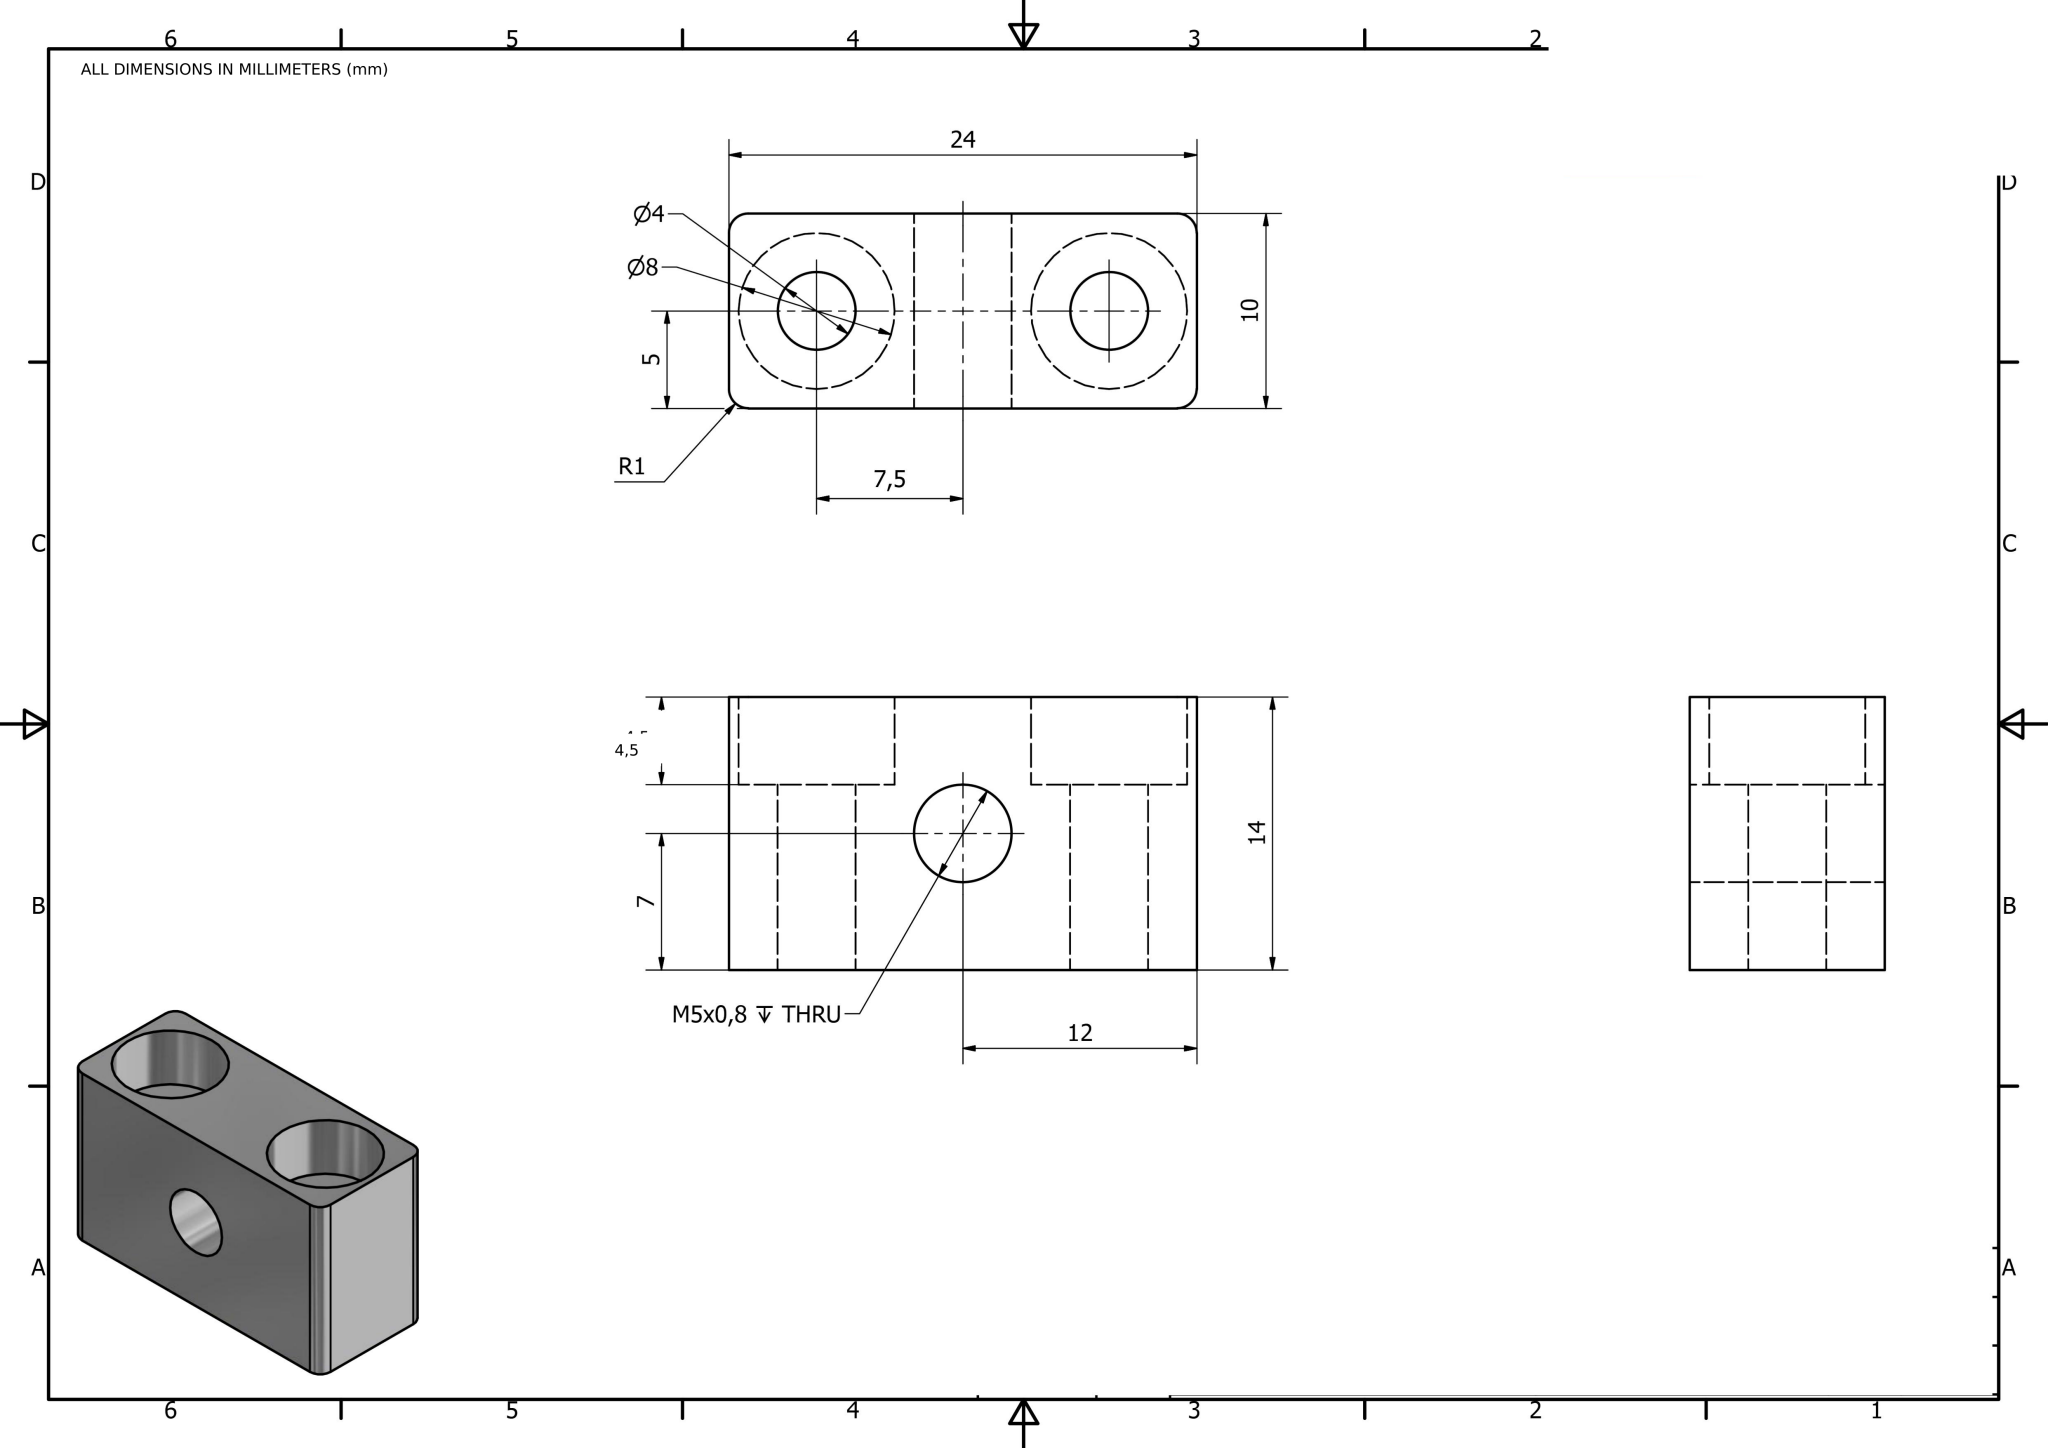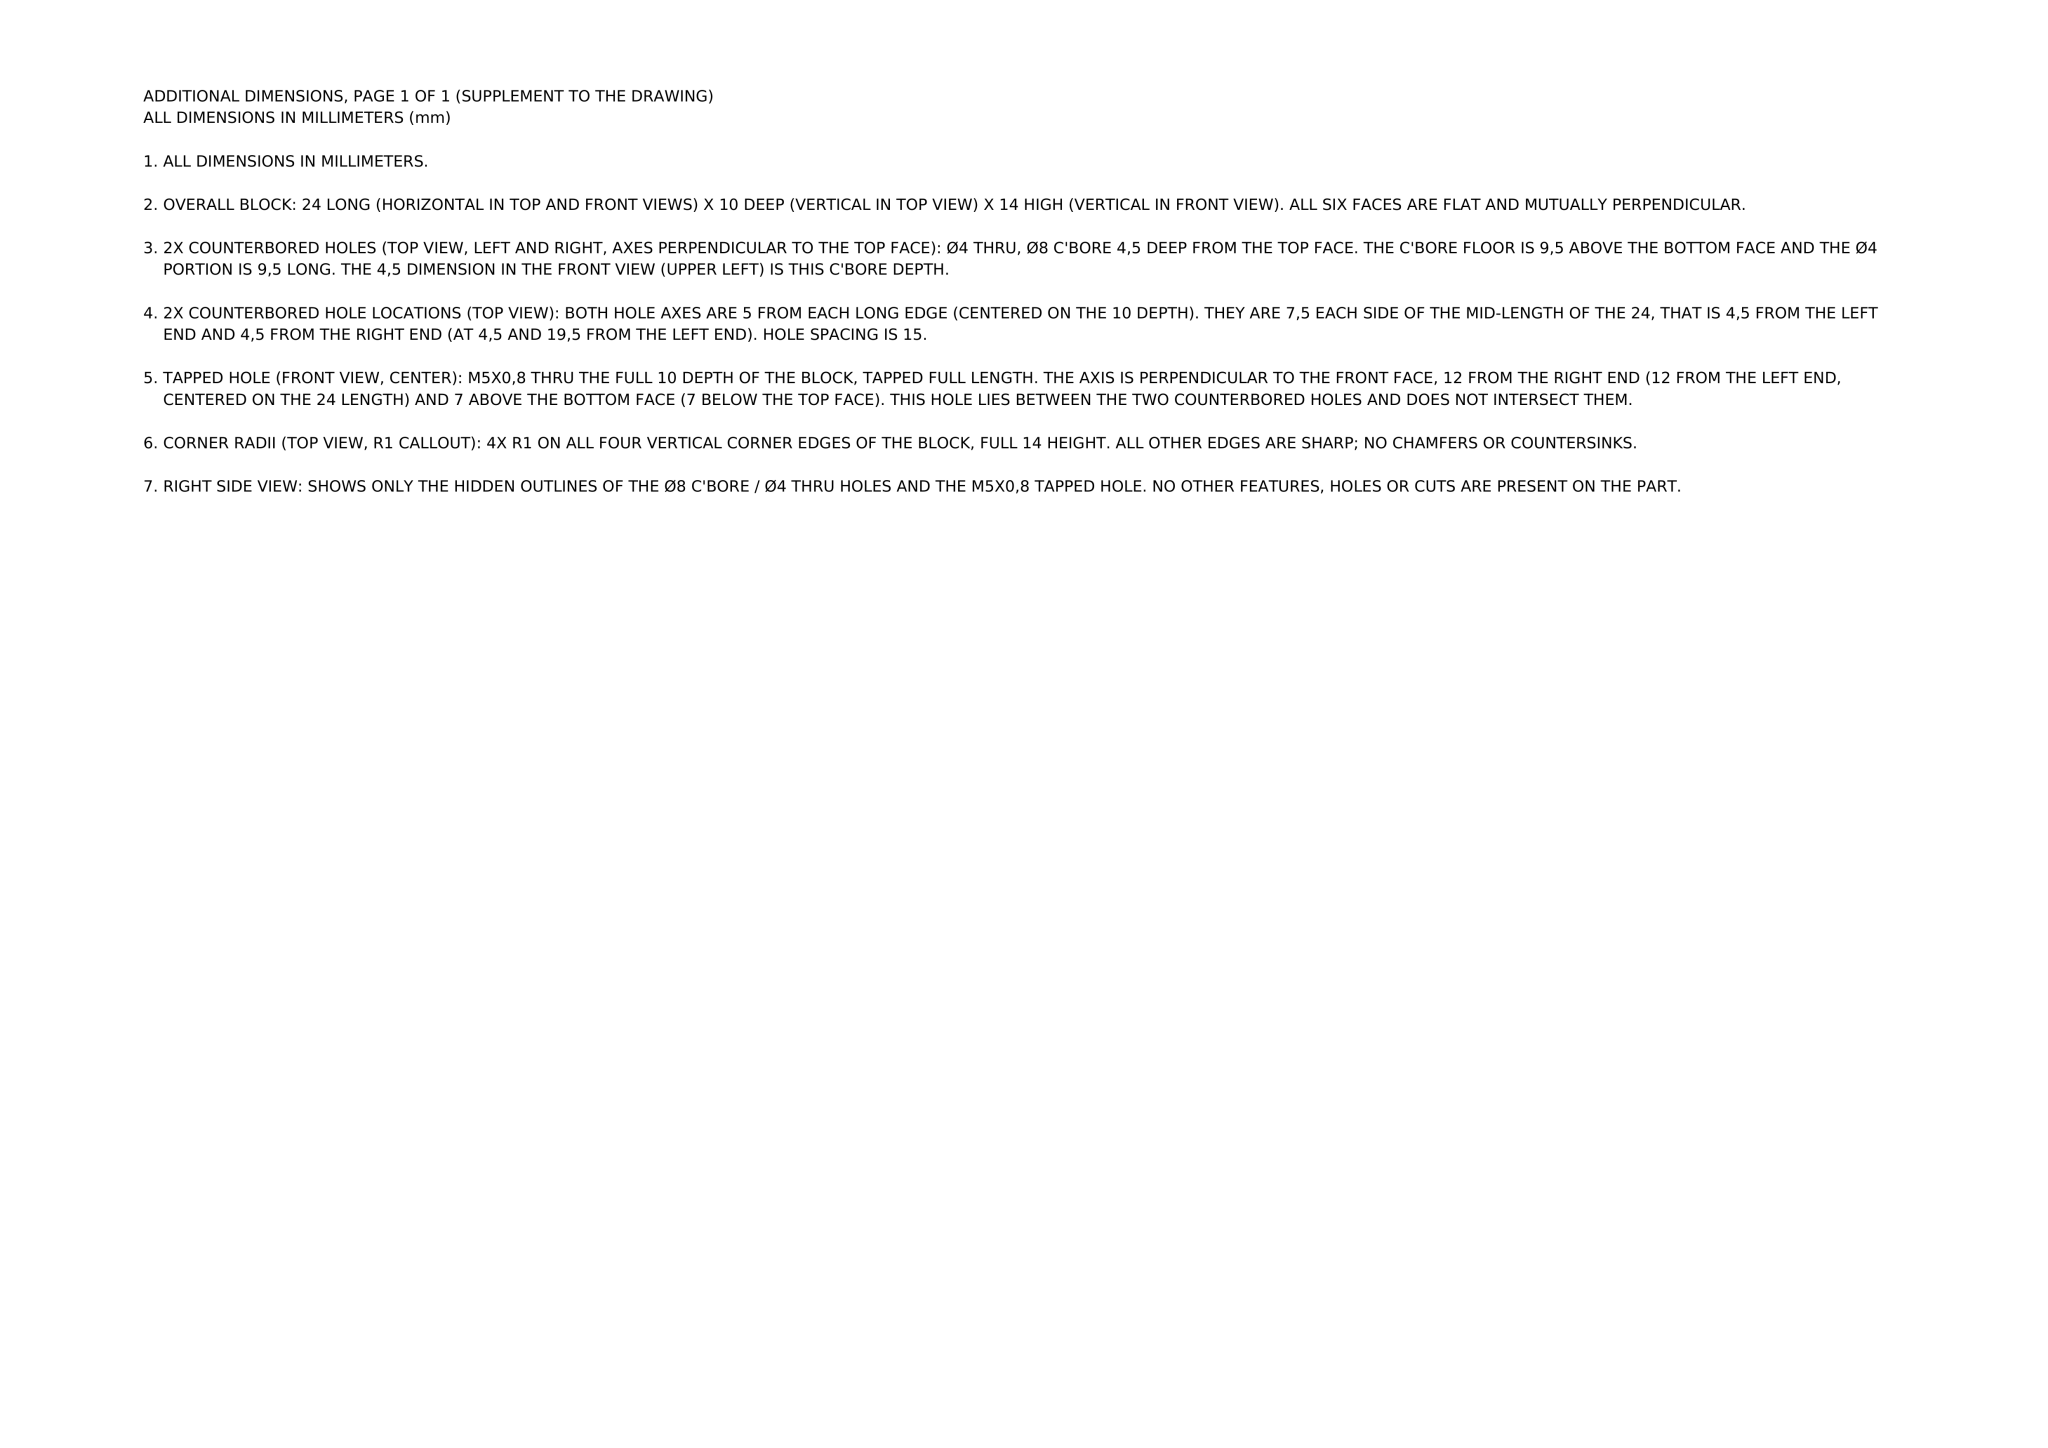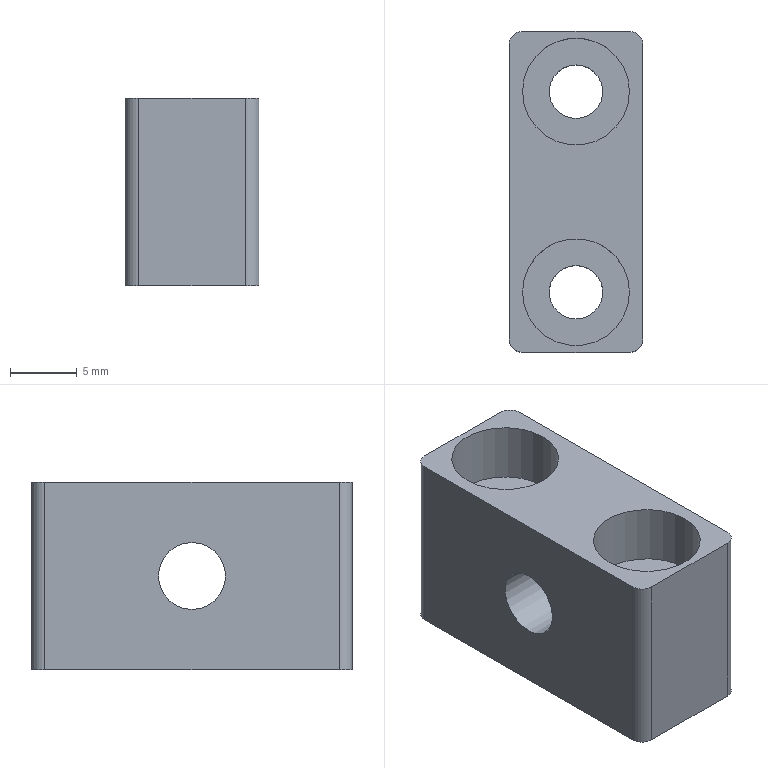Part | NX | mm | 1 solid | 17 faces | box 10 x 24 x 14 mm | volume 2460 mm3 | cylinder 9 | plane 8 | commonest cylinder face diameters 2 x4 8 x2 4 x2 5 x1
STEP:
#1=COLOUR_RGB('',0.9569,0.9569,0.9569);
#2=FILL_AREA_STYLE_COLOUR('',#1);
#3=FILL_AREA_STYLE('',(#2));
#4=SURFACE_STYLE_FILL_AREA(#3);
#5=SURFACE_SIDE_STYLE('',(#4));
#6=SURFACE_STYLE_USAGE(.BOTH.,#5);
#7=PRESENTATION_STYLE_ASSIGNMENT((#6));
#8=CARTESIAN_POINT('',(183.489,223.02,108.));
#9=VERTEX_POINT('',#8);
#10=CARTESIAN_POINT('',(182.489,222.02,108.));
#11=VERTEX_POINT('',#10);
#12=CARTESIAN_POINT('',(182.489,223.02,108.));
#13=DIRECTION('',(0.,0.,-1.));
#14=DIRECTION('',(0.7071,-0.7071,0.));
#15=AXIS2_PLACEMENT_3D('',#12,#13,#14);
#16=CIRCLE('',#15,1.);
#17=EDGE_CURVE('',#9,#11,#16,.T.);
#18=ORIENTED_EDGE('',*,*,#17,.T.);
#19=CARTESIAN_POINT('',(182.489,222.02,94.));
#20=VERTEX_POINT('',#19);
#21=CARTESIAN_POINT('',(182.489,222.02,94.));
#22=DIRECTION('',(0.,0.,-1.));
#23=VECTOR('',#22,1.);
#24=LINE('',#21,#23);
#25=EDGE_CURVE('',#11,#20,#24,.T.);
#26=ORIENTED_EDGE('',*,*,#25,.T.);
#27=CARTESIAN_POINT('',(183.489,223.02,94.));
#28=VERTEX_POINT('',#27);
#29=CARTESIAN_POINT('',(182.489,223.02,94.));
#30=DIRECTION('',(-0.,-0.,1.));
#31=DIRECTION('',(0.7071,-0.7071,0.));
#32=AXIS2_PLACEMENT_3D('',#29,#30,#31);
#33=CIRCLE('',#32,1.);
#34=EDGE_CURVE('',#20,#28,#33,.T.);
#35=ORIENTED_EDGE('',*,*,#34,.T.);
#36=CARTESIAN_POINT('',(183.489,223.02,94.));
#37=DIRECTION('',(0.,0.,1.));
#38=VECTOR('',#37,1.);
#39=LINE('',#36,#38);
#40=EDGE_CURVE('',#28,#9,#39,.T.);
#41=ORIENTED_EDGE('',*,*,#40,.T.);
#42=EDGE_LOOP('',(#18,#26,#35,#41));
#43=FACE_OUTER_BOUND('',#42,.T.);
#44=CARTESIAN_POINT('',(182.489,223.02,94.));
#45=DIRECTION('',(0.,0.,1.));
#46=DIRECTION('',(0.7071,-0.7071,0.));
#47=AXIS2_PLACEMENT_3D('',#44,#45,#46);
#48=CYLINDRICAL_SURFACE('',#47,1.);
#49=ADVANCED_FACE('',(#43),#48,.T.);
#50=STYLED_ITEM('',(#7),#49);
#51=ORIENTED_EDGE('',*,*,#34,.F.);
#52=CARTESIAN_POINT('',(174.489,222.02,94.));
#53=VERTEX_POINT('',#52);
#54=CARTESIAN_POINT('',(183.489,222.02,94.));
#55=DIRECTION('',(-1.,0.,0.));
#56=VECTOR('',#55,1.);
#57=LINE('',#54,#56);
#58=EDGE_CURVE('',#20,#53,#57,.T.);
#59=ORIENTED_EDGE('',*,*,#58,.T.);
#60=CARTESIAN_POINT('',(173.489,223.02,94.));
#61=VERTEX_POINT('',#60);
#62=CARTESIAN_POINT('',(174.489,223.02,94.));
#63=DIRECTION('',(-0.,-0.,1.));
#64=DIRECTION('',(-0.7071,-0.7071,-0.));
#65=AXIS2_PLACEMENT_3D('',#62,#63,#64);
#66=CIRCLE('',#65,1.);
#67=EDGE_CURVE('',#61,#53,#66,.T.);
#68=ORIENTED_EDGE('',*,*,#67,.F.);
#69=CARTESIAN_POINT('',(173.489,245.02,94.));
#70=VERTEX_POINT('',#69);
#71=CARTESIAN_POINT('',(173.489,222.02,94.));
#72=DIRECTION('',(0.,1.,0.));
#73=VECTOR('',#72,1.);
#74=LINE('',#71,#73);
#75=EDGE_CURVE('',#61,#70,#74,.T.);
#76=ORIENTED_EDGE('',*,*,#75,.T.);
#77=CARTESIAN_POINT('',(174.489,246.02,94.));
#78=VERTEX_POINT('',#77);
#79=CARTESIAN_POINT('',(174.489,245.02,94.));
#80=DIRECTION('',(-0.,-0.,1.));
#81=DIRECTION('',(-0.7071,0.7071,-0.));
#82=AXIS2_PLACEMENT_3D('',#79,#80,#81);
#83=CIRCLE('',#82,1.);
#84=EDGE_CURVE('',#78,#70,#83,.T.);
#85=ORIENTED_EDGE('',*,*,#84,.F.);
#86=CARTESIAN_POINT('',(182.489,246.02,94.));
#87=VERTEX_POINT('',#86);
#88=CARTESIAN_POINT('',(173.489,246.02,94.));
#89=DIRECTION('',(1.,0.,0.));
#90=VECTOR('',#89,1.);
#91=LINE('',#88,#90);
#92=EDGE_CURVE('',#78,#87,#91,.T.);
#93=ORIENTED_EDGE('',*,*,#92,.T.);
#94=CARTESIAN_POINT('',(183.489,245.02,94.));
#95=VERTEX_POINT('',#94);
#96=CARTESIAN_POINT('',(182.489,245.02,94.));
#97=DIRECTION('',(-0.,-0.,1.));
#98=DIRECTION('',(0.7071,0.7071,0.));
#99=AXIS2_PLACEMENT_3D('',#96,#97,#98);
#100=CIRCLE('',#99,1.);
#101=EDGE_CURVE('',#95,#87,#100,.T.);
#102=ORIENTED_EDGE('',*,*,#101,.F.);
#103=CARTESIAN_POINT('',(183.489,246.02,94.));
#104=DIRECTION('',(0.,-1.,0.));
#105=VECTOR('',#104,1.);
#106=LINE('',#103,#105);
#107=EDGE_CURVE('',#95,#28,#106,.T.);
#108=ORIENTED_EDGE('',*,*,#107,.T.);
#109=EDGE_LOOP('',(#51,#59,#68,#76,#85,#93,#102,#108));
#110=FACE_OUTER_BOUND('',#109,.T.);
#111=CARTESIAN_POINT('',(178.489,228.52,94.));
#112=VERTEX_POINT('',#111);
#113=CARTESIAN_POINT('',(178.489,226.52,94.));
#114=DIRECTION('',(-0.,-0.,1.));
#115=DIRECTION('',(0.,-1.,-0.));
#116=AXIS2_PLACEMENT_3D('',#113,#114,#115);
#117=CIRCLE('',#116,2.);
#118=EDGE_CURVE('',#112,#112,#117,.T.);
#119=ORIENTED_EDGE('',*,*,#118,.T.);
#120=EDGE_LOOP('',(#119));
#121=FACE_BOUND('',#120,.T.);
#122=CARTESIAN_POINT('',(178.489,243.52,94.));
#123=VERTEX_POINT('',#122);
#124=CARTESIAN_POINT('',(178.489,241.52,94.));
#125=DIRECTION('',(-0.,-0.,1.));
#126=DIRECTION('',(0.,-1.,-0.));
#127=AXIS2_PLACEMENT_3D('',#124,#125,#126);
#128=CIRCLE('',#127,2.);
#129=EDGE_CURVE('',#123,#123,#128,.T.);
#130=ORIENTED_EDGE('',*,*,#129,.T.);
#131=EDGE_LOOP('',(#130));
#132=FACE_BOUND('',#131,.T.);
#133=CARTESIAN_POINT('',(178.489,234.02,94.));
#134=DIRECTION('',(-0.,-0.,1.));
#135=DIRECTION('',(1.,0.,0.));
#136=AXIS2_PLACEMENT_3D('',#133,#134,#135);
#137=PLANE('',#136);
#138=ADVANCED_FACE('',(#110,#121,#132),#137,.F.);
#139=STYLED_ITEM('',(#7),#138);
#140=ORIENTED_EDGE('',*,*,#25,.F.);
#141=CARTESIAN_POINT('',(174.489,222.02,108.));
#142=VERTEX_POINT('',#141);
#143=CARTESIAN_POINT('',(183.489,222.02,108.));
#144=DIRECTION('',(-1.,0.,0.));
#145=VECTOR('',#144,1.);
#146=LINE('',#143,#145);
#147=EDGE_CURVE('',#11,#142,#146,.T.);
#148=ORIENTED_EDGE('',*,*,#147,.T.);
#149=CARTESIAN_POINT('',(174.489,222.02,94.));
#150=DIRECTION('',(0.,0.,1.));
#151=VECTOR('',#150,1.);
#152=LINE('',#149,#151);
#153=EDGE_CURVE('',#53,#142,#152,.T.);
#154=ORIENTED_EDGE('',*,*,#153,.F.);
#155=ORIENTED_EDGE('',*,*,#58,.F.);
#156=EDGE_LOOP('',(#140,#148,#154,#155));
#157=FACE_OUTER_BOUND('',#156,.T.);
#158=CARTESIAN_POINT('',(178.489,222.02,94.));
#159=DIRECTION('',(0.,-1.,0.));
#160=DIRECTION('',(1.,0.,0.));
#161=AXIS2_PLACEMENT_3D('',#158,#159,#160);
#162=PLANE('',#161);
#163=ADVANCED_FACE('',(#157),#162,.T.);
#164=STYLED_ITEM('',(#7),#163);
#165=CARTESIAN_POINT('',(173.489,223.02,108.));
#166=VERTEX_POINT('',#165);
#167=CARTESIAN_POINT('',(174.489,223.02,108.));
#168=DIRECTION('',(0.,0.,-1.));
#169=DIRECTION('',(-0.7071,-0.7071,-0.));
#170=AXIS2_PLACEMENT_3D('',#167,#168,#169);
#171=CIRCLE('',#170,1.);
#172=EDGE_CURVE('',#142,#166,#171,.T.);
#173=ORIENTED_EDGE('',*,*,#172,.T.);
#174=CARTESIAN_POINT('',(173.489,223.02,94.));
#175=DIRECTION('',(0.,0.,-1.));
#176=VECTOR('',#175,1.);
#177=LINE('',#174,#176);
#178=EDGE_CURVE('',#166,#61,#177,.T.);
#179=ORIENTED_EDGE('',*,*,#178,.T.);
#180=ORIENTED_EDGE('',*,*,#67,.T.);
#181=ORIENTED_EDGE('',*,*,#153,.T.);
#182=EDGE_LOOP('',(#173,#179,#180,#181));
#183=FACE_OUTER_BOUND('',#182,.T.);
#184=CARTESIAN_POINT('',(174.489,223.02,94.));
#185=DIRECTION('',(0.,0.,1.));
#186=DIRECTION('',(-0.7071,-0.7071,0.));
#187=AXIS2_PLACEMENT_3D('',#184,#185,#186);
#188=CYLINDRICAL_SURFACE('',#187,1.);
#189=ADVANCED_FACE('',(#183),#188,.T.);
#190=STYLED_ITEM('',(#7),#189);
#191=CARTESIAN_POINT('',(182.489,246.02,108.));
#192=VERTEX_POINT('',#191);
#193=CARTESIAN_POINT('',(183.489,245.02,108.));
#194=VERTEX_POINT('',#193);
#195=CARTESIAN_POINT('',(182.489,245.02,108.));
#196=DIRECTION('',(0.,0.,-1.));
#197=DIRECTION('',(0.7071,0.7071,0.));
#198=AXIS2_PLACEMENT_3D('',#195,#196,#197);
#199=CIRCLE('',#198,1.);
#200=EDGE_CURVE('',#192,#194,#199,.T.);
#201=ORIENTED_EDGE('',*,*,#200,.T.);
#202=CARTESIAN_POINT('',(183.489,245.02,94.));
#203=DIRECTION('',(0.,0.,-1.));
#204=VECTOR('',#203,1.);
#205=LINE('',#202,#204);
#206=EDGE_CURVE('',#194,#95,#205,.T.);
#207=ORIENTED_EDGE('',*,*,#206,.T.);
#208=ORIENTED_EDGE('',*,*,#101,.T.);
#209=CARTESIAN_POINT('',(182.489,246.02,94.));
#210=DIRECTION('',(0.,0.,1.));
#211=VECTOR('',#210,1.);
#212=LINE('',#209,#211);
#213=EDGE_CURVE('',#87,#192,#212,.T.);
#214=ORIENTED_EDGE('',*,*,#213,.T.);
#215=EDGE_LOOP('',(#201,#207,#208,#214));
#216=FACE_OUTER_BOUND('',#215,.T.);
#217=CARTESIAN_POINT('',(182.489,245.02,94.));
#218=DIRECTION('',(0.,0.,1.));
#219=DIRECTION('',(0.7071,0.7071,0.));
#220=AXIS2_PLACEMENT_3D('',#217,#218,#219);
#221=CYLINDRICAL_SURFACE('',#220,1.);
#222=ADVANCED_FACE('',(#216),#221,.T.);
#223=STYLED_ITEM('',(#7),#222);
#224=ORIENTED_EDGE('',*,*,#213,.F.);
#225=ORIENTED_EDGE('',*,*,#92,.F.);
#226=CARTESIAN_POINT('',(174.489,246.02,108.));
#227=VERTEX_POINT('',#226);
#228=CARTESIAN_POINT('',(174.489,246.02,94.));
#229=DIRECTION('',(0.,0.,-1.));
#230=VECTOR('',#229,1.);
#231=LINE('',#228,#230);
#232=EDGE_CURVE('',#227,#78,#231,.T.);
#233=ORIENTED_EDGE('',*,*,#232,.F.);
#234=CARTESIAN_POINT('',(173.489,246.02,108.));
#235=DIRECTION('',(1.,0.,0.));
#236=VECTOR('',#235,1.);
#237=LINE('',#234,#236);
#238=EDGE_CURVE('',#227,#192,#237,.T.);
#239=ORIENTED_EDGE('',*,*,#238,.T.);
#240=EDGE_LOOP('',(#224,#225,#233,#239));
#241=FACE_OUTER_BOUND('',#240,.T.);
#242=CARTESIAN_POINT('',(178.489,246.02,94.));
#243=DIRECTION('',(0.,1.,0.));
#244=DIRECTION('',(-1.,0.,0.));
#245=AXIS2_PLACEMENT_3D('',#242,#243,#244);
#246=PLANE('',#245);
#247=ADVANCED_FACE('',(#241),#246,.T.);
#248=STYLED_ITEM('',(#7),#247);
#249=CARTESIAN_POINT('',(173.489,245.02,108.));
#250=VERTEX_POINT('',#249);
#251=CARTESIAN_POINT('',(174.489,245.02,108.));
#252=DIRECTION('',(0.,0.,-1.));
#253=DIRECTION('',(-0.7071,0.7071,-0.));
#254=AXIS2_PLACEMENT_3D('',#251,#252,#253);
#255=CIRCLE('',#254,1.);
#256=EDGE_CURVE('',#250,#227,#255,.T.);
#257=ORIENTED_EDGE('',*,*,#256,.T.);
#258=ORIENTED_EDGE('',*,*,#232,.T.);
#259=ORIENTED_EDGE('',*,*,#84,.T.);
#260=CARTESIAN_POINT('',(173.489,245.02,94.));
#261=DIRECTION('',(0.,0.,1.));
#262=VECTOR('',#261,1.);
#263=LINE('',#260,#262);
#264=EDGE_CURVE('',#70,#250,#263,.T.);
#265=ORIENTED_EDGE('',*,*,#264,.T.);
#266=EDGE_LOOP('',(#257,#258,#259,#265));
#267=FACE_OUTER_BOUND('',#266,.T.);
#268=CARTESIAN_POINT('',(174.489,245.02,94.));
#269=DIRECTION('',(0.,0.,1.));
#270=DIRECTION('',(-0.7071,0.7071,0.));
#271=AXIS2_PLACEMENT_3D('',#268,#269,#270);
#272=CYLINDRICAL_SURFACE('',#271,1.);
#273=ADVANCED_FACE('',(#267),#272,.T.);
#274=STYLED_ITEM('',(#7),#273);
#275=CARTESIAN_POINT('',(182.489,226.52,103.5));
#276=VERTEX_POINT('',#275);
#277=CARTESIAN_POINT('',(174.489,226.52,103.5));
#278=VERTEX_POINT('',#277);
#279=CARTESIAN_POINT('',(178.489,226.52,103.5));
#280=DIRECTION('',(0.,0.,-1.));
#281=DIRECTION('',(1.,0.,0.));
#282=AXIS2_PLACEMENT_3D('',#279,#280,#281);
#283=CIRCLE('',#282,4.);
#284=EDGE_CURVE('',#276,#278,#283,.T.);
#285=ORIENTED_EDGE('',*,*,#284,.F.);
#286=CARTESIAN_POINT('',(178.489,226.52,103.5));
#287=DIRECTION('',(0.,0.,-1.));
#288=DIRECTION('',(1.,0.,0.));
#289=AXIS2_PLACEMENT_3D('',#286,#287,#288);
#290=CIRCLE('',#289,4.);
#291=EDGE_CURVE('',#278,#276,#290,.T.);
#292=ORIENTED_EDGE('',*,*,#291,.F.);
#293=EDGE_LOOP('',(#285,#292));
#294=FACE_OUTER_BOUND('',#293,.T.);
#295=CARTESIAN_POINT('',(178.489,228.52,103.5));
#296=VERTEX_POINT('',#295);
#297=CARTESIAN_POINT('',(178.489,226.52,103.5));
#298=DIRECTION('',(0.,0.,-1.));
#299=DIRECTION('',(0.,-1.,0.));
#300=AXIS2_PLACEMENT_3D('',#297,#298,#299);
#301=CIRCLE('',#300,2.);
#302=EDGE_CURVE('',#296,#296,#301,.T.);
#303=ORIENTED_EDGE('',*,*,#302,.T.);
#304=EDGE_LOOP('',(#303));
#305=FACE_BOUND('',#304,.T.);
#306=CARTESIAN_POINT('',(178.489,226.52,103.5));
#307=DIRECTION('',(0.,0.,-1.));
#308=DIRECTION('',(1.,0.,0.));
#309=AXIS2_PLACEMENT_3D('',#306,#307,#308);
#310=PLANE('',#309);
#311=ADVANCED_FACE('',(#294,#305),#310,.F.);
#312=STYLED_ITEM('',(#7),#311);
#313=CARTESIAN_POINT('',(174.489,226.52,108.));
#314=VERTEX_POINT('',#313);
#315=CARTESIAN_POINT('',(178.489,226.52,108.));
#316=DIRECTION('',(0.,0.,-1.));
#317=DIRECTION('',(1.,-0.,0.));
#318=AXIS2_PLACEMENT_3D('',#315,#316,#317);
#319=CIRCLE('',#318,4.);
#320=EDGE_CURVE('',#314,#314,#319,.T.);
#321=ORIENTED_EDGE('',*,*,#320,.F.);
#322=CARTESIAN_POINT('',(174.489,226.52,109.75));
#323=DIRECTION('',(0.,0.,-1.));
#324=VECTOR('',#323,4.);
#325=LINE('',#322,#324);
#326=EDGE_CURVE('',#314,#278,#325,.T.);
#327=ORIENTED_EDGE('',*,*,#326,.T.);
#328=ORIENTED_EDGE('',*,*,#291,.T.);
#329=ORIENTED_EDGE('',*,*,#284,.T.);
#330=ORIENTED_EDGE('',*,*,#326,.F.);
#331=EDGE_LOOP('',(#321,#327,#328,#329,#330));
#332=FACE_OUTER_BOUND('',#331,.T.);
#333=CARTESIAN_POINT('',(178.489,226.52,109.75));
#334=DIRECTION('',(0.,0.,-1.));
#335=DIRECTION('',(1.,0.,0.));
#336=AXIS2_PLACEMENT_3D('',#333,#334,#335);
#337=CYLINDRICAL_SURFACE('',#336,4.);
#338=ADVANCED_FACE('',(#332),#337,.F.);
#339=STYLED_ITEM('',(#7),#338);
#340=ORIENTED_EDGE('',*,*,#302,.F.);
#341=CARTESIAN_POINT('',(178.489,228.52,116.));
#342=DIRECTION('',(0.,0.,-1.));
#343=VECTOR('',#342,2.);
#344=LINE('',#341,#343);
#345=EDGE_CURVE('',#296,#112,#344,.T.);
#346=ORIENTED_EDGE('',*,*,#345,.T.);
#347=ORIENTED_EDGE('',*,*,#118,.F.);
#348=ORIENTED_EDGE('',*,*,#345,.F.);
#349=EDGE_LOOP('',(#340,#346,#347,#348));
#350=FACE_OUTER_BOUND('',#349,.T.);
#351=CARTESIAN_POINT('',(178.489,226.52,116.));
#352=DIRECTION('',(0.,0.,-1.));
#353=DIRECTION('',(0.,-1.,0.));
#354=AXIS2_PLACEMENT_3D('',#351,#352,#353);
#355=CYLINDRICAL_SURFACE('',#354,2.);
#356=ADVANCED_FACE('',(#350),#355,.F.);
#357=STYLED_ITEM('',(#7),#356);
#358=CARTESIAN_POINT('',(182.489,241.52,103.5));
#359=VERTEX_POINT('',#358);
#360=CARTESIAN_POINT('',(174.489,241.52,103.5));
#361=VERTEX_POINT('',#360);
#362=CARTESIAN_POINT('',(178.489,241.52,103.5));
#363=DIRECTION('',(0.,0.,-1.));
#364=DIRECTION('',(1.,0.,0.));
#365=AXIS2_PLACEMENT_3D('',#362,#363,#364);
#366=CIRCLE('',#365,4.);
#367=EDGE_CURVE('',#359,#361,#366,.T.);
#368=ORIENTED_EDGE('',*,*,#367,.F.);
#369=CARTESIAN_POINT('',(178.489,241.52,103.5));
#370=DIRECTION('',(0.,0.,-1.));
#371=DIRECTION('',(1.,0.,0.));
#372=AXIS2_PLACEMENT_3D('',#369,#370,#371);
#373=CIRCLE('',#372,4.);
#374=EDGE_CURVE('',#361,#359,#373,.T.);
#375=ORIENTED_EDGE('',*,*,#374,.F.);
#376=EDGE_LOOP('',(#368,#375));
#377=FACE_OUTER_BOUND('',#376,.T.);
#378=CARTESIAN_POINT('',(178.489,243.52,103.5));
#379=VERTEX_POINT('',#378);
#380=CARTESIAN_POINT('',(178.489,241.52,103.5));
#381=DIRECTION('',(0.,0.,-1.));
#382=DIRECTION('',(0.,-1.,0.));
#383=AXIS2_PLACEMENT_3D('',#380,#381,#382);
#384=CIRCLE('',#383,2.);
#385=EDGE_CURVE('',#379,#379,#384,.T.);
#386=ORIENTED_EDGE('',*,*,#385,.T.);
#387=EDGE_LOOP('',(#386));
#388=FACE_BOUND('',#387,.T.);
#389=CARTESIAN_POINT('',(178.489,241.52,103.5));
#390=DIRECTION('',(0.,0.,-1.));
#391=DIRECTION('',(1.,0.,0.));
#392=AXIS2_PLACEMENT_3D('',#389,#390,#391);
#393=PLANE('',#392);
#394=ADVANCED_FACE('',(#377,#388),#393,.F.);
#395=STYLED_ITEM('',(#7),#394);
#396=CARTESIAN_POINT('',(174.489,241.52,108.));
#397=VERTEX_POINT('',#396);
#398=CARTESIAN_POINT('',(178.489,241.52,108.));
#399=DIRECTION('',(0.,0.,-1.));
#400=DIRECTION('',(1.,-0.,0.));
#401=AXIS2_PLACEMENT_3D('',#398,#399,#400);
#402=CIRCLE('',#401,4.);
#403=EDGE_CURVE('',#397,#397,#402,.T.);
#404=ORIENTED_EDGE('',*,*,#403,.F.);
#405=CARTESIAN_POINT('',(174.489,241.52,109.75));
#406=DIRECTION('',(0.,0.,-1.));
#407=VECTOR('',#406,4.);
#408=LINE('',#405,#407);
#409=EDGE_CURVE('',#397,#361,#408,.T.);
#410=ORIENTED_EDGE('',*,*,#409,.T.);
#411=ORIENTED_EDGE('',*,*,#374,.T.);
#412=ORIENTED_EDGE('',*,*,#367,.T.);
#413=ORIENTED_EDGE('',*,*,#409,.F.);
#414=EDGE_LOOP('',(#404,#410,#411,#412,#413));
#415=FACE_OUTER_BOUND('',#414,.T.);
#416=CARTESIAN_POINT('',(178.489,241.52,109.75));
#417=DIRECTION('',(0.,0.,-1.));
#418=DIRECTION('',(1.,0.,0.));
#419=AXIS2_PLACEMENT_3D('',#416,#417,#418);
#420=CYLINDRICAL_SURFACE('',#419,4.);
#421=ADVANCED_FACE('',(#415),#420,.F.);
#422=STYLED_ITEM('',(#7),#421);
#423=ORIENTED_EDGE('',*,*,#385,.F.);
#424=CARTESIAN_POINT('',(178.489,243.52,116.));
#425=DIRECTION('',(0.,0.,-1.));
#426=VECTOR('',#425,2.);
#427=LINE('',#424,#426);
#428=EDGE_CURVE('',#379,#123,#427,.T.);
#429=ORIENTED_EDGE('',*,*,#428,.T.);
#430=ORIENTED_EDGE('',*,*,#129,.F.);
#431=ORIENTED_EDGE('',*,*,#428,.F.);
#432=EDGE_LOOP('',(#423,#429,#430,#431));
#433=FACE_OUTER_BOUND('',#432,.T.);
#434=CARTESIAN_POINT('',(178.489,241.52,116.));
#435=DIRECTION('',(0.,0.,-1.));
#436=DIRECTION('',(0.,-1.,0.));
#437=AXIS2_PLACEMENT_3D('',#434,#435,#436);
#438=CYLINDRICAL_SURFACE('',#437,2.);
#439=ADVANCED_FACE('',(#433),#438,.F.);
#440=STYLED_ITEM('',(#7),#439);
#441=CARTESIAN_POINT('',(173.489,234.02,98.5));
#442=VERTEX_POINT('',#441);
#443=CARTESIAN_POINT('',(173.489,234.02,101.));
#444=DIRECTION('',(1.,0.,0.));
#445=DIRECTION('',(0.,0.,1.));
#446=AXIS2_PLACEMENT_3D('',#443,#444,#445);
#447=CIRCLE('',#446,2.5);
#448=EDGE_CURVE('',#442,#442,#447,.T.);
#449=ORIENTED_EDGE('',*,*,#448,.F.);
#450=CARTESIAN_POINT('',(183.489,234.02,98.5));
#451=VERTEX_POINT('',#450);
#452=CARTESIAN_POINT('',(146.789,234.02,98.5));
#453=DIRECTION('',(1.,0.,0.));
#454=VECTOR('',#453,2.5);
#455=LINE('',#452,#454);
#456=EDGE_CURVE('',#442,#451,#455,.T.);
#457=ORIENTED_EDGE('',*,*,#456,.T.);
#458=CARTESIAN_POINT('',(183.489,234.02,101.));
#459=DIRECTION('',(-1.,0.,0.));
#460=DIRECTION('',(0.,0.,1.));
#461=AXIS2_PLACEMENT_3D('',#458,#459,#460);
#462=CIRCLE('',#461,2.5);
#463=EDGE_CURVE('',#451,#451,#462,.T.);
#464=ORIENTED_EDGE('',*,*,#463,.F.);
#465=ORIENTED_EDGE('',*,*,#456,.F.);
#466=EDGE_LOOP('',(#449,#457,#464,#465));
#467=FACE_OUTER_BOUND('',#466,.T.);
#468=CARTESIAN_POINT('',(146.789,234.02,101.));
#469=DIRECTION('',(1.,0.,0.));
#470=DIRECTION('',(0.,0.,1.));
#471=AXIS2_PLACEMENT_3D('',#468,#469,#470);
#472=CYLINDRICAL_SURFACE('',#471,2.5);
#473=ADVANCED_FACE('',(#467),#472,.F.);
#474=STYLED_ITEM('',(#7),#473);
#475=ORIENTED_EDGE('',*,*,#178,.F.);
#476=CARTESIAN_POINT('',(173.489,222.02,108.));
#477=DIRECTION('',(0.,1.,0.));
#478=VECTOR('',#477,1.);
#479=LINE('',#476,#478);
#480=EDGE_CURVE('',#166,#250,#479,.T.);
#481=ORIENTED_EDGE('',*,*,#480,.T.);
#482=ORIENTED_EDGE('',*,*,#264,.F.);
#483=ORIENTED_EDGE('',*,*,#75,.F.);
#484=EDGE_LOOP('',(#475,#481,#482,#483));
#485=FACE_OUTER_BOUND('',#484,.T.);
#486=ORIENTED_EDGE('',*,*,#448,.T.);
#487=EDGE_LOOP('',(#486));
#488=FACE_BOUND('',#487,.T.);
#489=CARTESIAN_POINT('',(173.489,234.02,94.));
#490=DIRECTION('',(-1.,0.,0.));
#491=DIRECTION('',(0.,-1.,0.));
#492=AXIS2_PLACEMENT_3D('',#489,#490,#491);
#493=PLANE('',#492);
#494=ADVANCED_FACE('',(#485,#488),#493,.T.);
#495=STYLED_ITEM('',(#7),#494);
#496=ORIENTED_EDGE('',*,*,#40,.F.);
#497=ORIENTED_EDGE('',*,*,#107,.F.);
#498=ORIENTED_EDGE('',*,*,#206,.F.);
#499=CARTESIAN_POINT('',(183.489,246.02,108.));
#500=DIRECTION('',(0.,-1.,0.));
#501=VECTOR('',#500,1.);
#502=LINE('',#499,#501);
#503=EDGE_CURVE('',#194,#9,#502,.T.);
#504=ORIENTED_EDGE('',*,*,#503,.T.);
#505=EDGE_LOOP('',(#496,#497,#498,#504));
#506=FACE_OUTER_BOUND('',#505,.T.);
#507=ORIENTED_EDGE('',*,*,#463,.T.);
#508=EDGE_LOOP('',(#507));
#509=FACE_BOUND('',#508,.T.);
#510=CARTESIAN_POINT('',(183.489,234.02,94.));
#511=DIRECTION('',(1.,0.,0.));
#512=DIRECTION('',(0.,1.,0.));
#513=AXIS2_PLACEMENT_3D('',#510,#511,#512);
#514=PLANE('',#513);
#515=ADVANCED_FACE('',(#506,#509),#514,.T.);
#516=STYLED_ITEM('',(#7),#515);
#517=ORIENTED_EDGE('',*,*,#17,.F.);
#518=ORIENTED_EDGE('',*,*,#503,.F.);
#519=ORIENTED_EDGE('',*,*,#200,.F.);
#520=ORIENTED_EDGE('',*,*,#238,.F.);
#521=ORIENTED_EDGE('',*,*,#256,.F.);
#522=ORIENTED_EDGE('',*,*,#480,.F.);
#523=ORIENTED_EDGE('',*,*,#172,.F.);
#524=ORIENTED_EDGE('',*,*,#147,.F.);
#525=EDGE_LOOP('',(#517,#518,#519,#520,#521,#522,#523,#524));
#526=FACE_OUTER_BOUND('',#525,.T.);
#527=ORIENTED_EDGE('',*,*,#320,.T.);
#528=EDGE_LOOP('',(#527));
#529=FACE_BOUND('',#528,.T.);
#530=ORIENTED_EDGE('',*,*,#403,.T.);
#531=EDGE_LOOP('',(#530));
#532=FACE_BOUND('',#531,.T.);
#533=CARTESIAN_POINT('',(178.489,234.02,108.));
#534=DIRECTION('',(-0.,-0.,1.));
#535=DIRECTION('',(1.,0.,0.));
#536=AXIS2_PLACEMENT_3D('',#533,#534,#535);
#537=PLANE('',#536);
#538=ADVANCED_FACE('',(#526,#529,#532),#537,.T.);
#539=STYLED_ITEM('',(#7),#538);
#540=COLOUR_RGB('',0.9412,0.6275,0.4314);
#541=FILL_AREA_STYLE_COLOUR('',#540);
#542=FILL_AREA_STYLE('',(#541));
#543=SURFACE_STYLE_FILL_AREA(#542);
#544=SURFACE_SIDE_STYLE('',(#543));
#545=SURFACE_STYLE_USAGE(.BOTH.,#544);
#546=PRESENTATION_STYLE_ASSIGNMENT((#545));
#547=CLOSED_SHELL('',(#49,#138,#163,#189,#222,#247,#273,#311,#338,#356,#394,#421,#439,#473,#494,#515,#538));
#548=MANIFOLD_SOLID_BREP('',#547);
#549=STYLED_ITEM('',(#546),#548);
#550=(LENGTH_UNIT()NAMED_UNIT(*)SI_UNIT(.MILLI.,.METRE.));
#551=UNCERTAINTY_MEASURE_WITH_UNIT(LENGTH_MEASURE(0.01),#550,'','');
#552=(NAMED_UNIT(*)PLANE_ANGLE_UNIT()SI_UNIT($,.RADIAN.));
#553=(NAMED_UNIT(*)SI_UNIT($,.STERADIAN.)SOLID_ANGLE_UNIT());
#554=(GEOMETRIC_REPRESENTATION_CONTEXT(3)GLOBAL_UNCERTAINTY_ASSIGNED_CONTEXT((#551))GLOBAL_UNIT_ASSIGNED_CONTEXT((#550,#552,#553))REPRESENTATION_CONTEXT('',''));
#555=MECHANICAL_DESIGN_GEOMETRIC_PRESENTATION_REPRESENTATION('',(#50,#139,#164,#190,#223,#248,#274,#312,#339,#357,#395,#422,#440,#474,#495,#516,#539,#549),#554);
#556=CARTESIAN_POINT('',(0.,0.,0.));
#557=DIRECTION('',(0.,0.,1.));
#558=DIRECTION('',(1.,0.,0.));
#559=AXIS2_PLACEMENT_3D('',#556,#557,#558);
#560=UNCERTAINTY_MEASURE_WITH_UNIT(LENGTH_MEASURE(0.01),#550,'','');
#561=(GEOMETRIC_REPRESENTATION_CONTEXT(3)GLOBAL_UNCERTAINTY_ASSIGNED_CONTEXT((#560))GLOBAL_UNIT_ASSIGNED_CONTEXT((#550,#552,#553))REPRESENTATION_CONTEXT('',''));
#562=SHAPE_REPRESENTATION('',(#559),#561);
#563=ADVANCED_BREP_SHAPE_REPRESENTATION('',(#548),#561);
#564=SHAPE_REPRESENTATION_RELATIONSHIP('','',#562,#563);
#565=DESCRIPTIVE_REPRESENTATION_ITEM('','');
#566=REPRESENTATION('',(#565),#561);
#567=(MASS_UNIT()NAMED_UNIT(*)SI_UNIT($,.GRAM.));
#568=DERIVED_UNIT_ELEMENT(#567,1.);
#569=(LENGTH_UNIT()NAMED_UNIT(*)SI_UNIT(.CENTI.,.METRE.));
#570=DERIVED_UNIT_ELEMENT(#569,3.);
#571=DERIVED_UNIT((#568,#570));
#572=MEASURE_REPRESENTATION_ITEM('',POSITIVE_RATIO_MEASURE(1.),#571);
#573=REPRESENTATION('',(#572),#561);
#574=COLOUR_RGB('',0.749,0.749,0.749);
#575=FILL_AREA_STYLE_COLOUR('',#574);
#576=FILL_AREA_STYLE('',(#575));
#577=SURFACE_STYLE_FILL_AREA(#576);
#578=SURFACE_SIDE_STYLE('',(#577));
#579=SURFACE_STYLE_USAGE(.BOTH.,#578);
#580=PRESENTATION_STYLE_ASSIGNMENT((#579));